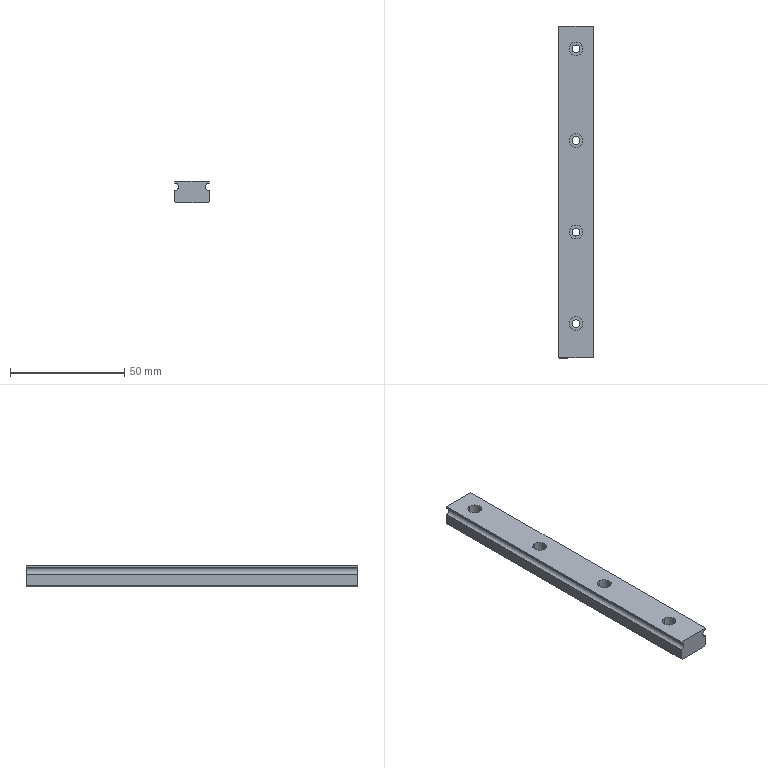Component | SolidWorks | 1-16-1 | 1 solid | 33 faces | box 15 x 145 x 9.5 mm | volume 18700 mm3 | cylinder 19 | plane 14 | commonest cylinder face diameters 6 x8 3.5 x8 3.28 x3
STEP:
#1=CARTESIAN_POINT('',(-4.34,3.239,-0.7858));
#2=VERTEX_POINT('',#1);
#3=CARTESIAN_POINT('',(-4.34,3.475,-0.7858));
#4=VERTEX_POINT('',#3);
#5=CARTESIAN_POINT('',(-4.34,3.357,-0.7858));
#6=DIRECTION('',(0.,0.,-1.));
#7=DIRECTION('',(0.,1.,0.));
#8=AXIS2_PLACEMENT_3D('',#5,#6,#7);
#9=CIRCLE('',#8,0.1181);
#10=EDGE_CURVE('',#2,#4,#9,.T.);
#11=ORIENTED_EDGE('',*,*,#10,.F.);
#12=CARTESIAN_POINT('',(-4.34,3.239,-0.963));
#13=VERTEX_POINT('',#12);
#14=CARTESIAN_POINT('',(-4.34,3.239,-0.8744));
#15=DIRECTION('',(0.,0.,-1.));
#16=VECTOR('',#15,39.37);
#17=LINE('',#14,#16);
#18=EDGE_CURVE('',#2,#13,#17,.T.);
#19=ORIENTED_EDGE('',*,*,#18,.T.);
#20=CARTESIAN_POINT('',(-4.34,3.475,-0.963));
#21=VERTEX_POINT('',#20);
#22=CARTESIAN_POINT('',(-4.34,3.357,-0.963));
#23=DIRECTION('',(-0.,-0.,1.));
#24=DIRECTION('',(0.,1.,0.));
#25=AXIS2_PLACEMENT_3D('',#22,#23,#24);
#26=CIRCLE('',#25,0.1181);
#27=EDGE_CURVE('',#21,#13,#26,.T.);
#28=ORIENTED_EDGE('',*,*,#27,.F.);
#29=CARTESIAN_POINT('',(-4.34,3.475,-0.8744));
#30=DIRECTION('',(0.,0.,-1.));
#31=VECTOR('',#30,39.37);
#32=LINE('',#29,#31);
#33=EDGE_CURVE('',#4,#21,#32,.T.);
#34=ORIENTED_EDGE('',*,*,#33,.F.);
#35=EDGE_LOOP('',(#11,#19,#28,#34));
#36=FACE_OUTER_BOUND('',#35,.T.);
#37=CARTESIAN_POINT('',(-4.34,3.357,-0.8744));
#38=DIRECTION('',(0.,0.,-1.));
#39=DIRECTION('',(0.,1.,0.));
#40=AXIS2_PLACEMENT_3D('',#37,#38,#39);
#41=CYLINDRICAL_SURFACE('',#40,0.1181);
#42=ADVANCED_FACE('',(#36),#41,.F.);
#43=CARTESIAN_POINT('',(-4.34,1.664,-0.7858));
#44=VERTEX_POINT('',#43);
#45=CARTESIAN_POINT('',(-4.34,1.9,-0.7858));
#46=VERTEX_POINT('',#45);
#47=CARTESIAN_POINT('',(-4.34,1.782,-0.7858));
#48=DIRECTION('',(0.,0.,-1.));
#49=DIRECTION('',(0.,1.,0.));
#50=AXIS2_PLACEMENT_3D('',#47,#48,#49);
#51=CIRCLE('',#50,0.1181);
#52=EDGE_CURVE('',#44,#46,#51,.T.);
#53=ORIENTED_EDGE('',*,*,#52,.F.);
#54=CARTESIAN_POINT('',(-4.34,1.664,-0.963));
#55=VERTEX_POINT('',#54);
#56=CARTESIAN_POINT('',(-4.34,1.664,-0.8744));
#57=DIRECTION('',(0.,0.,-1.));
#58=VECTOR('',#57,39.37);
#59=LINE('',#56,#58);
#60=EDGE_CURVE('',#44,#55,#59,.T.);
#61=ORIENTED_EDGE('',*,*,#60,.T.);
#62=CARTESIAN_POINT('',(-4.34,1.9,-0.963));
#63=VERTEX_POINT('',#62);
#64=CARTESIAN_POINT('',(-4.34,1.782,-0.963));
#65=DIRECTION('',(-0.,-0.,1.));
#66=DIRECTION('',(0.,1.,0.));
#67=AXIS2_PLACEMENT_3D('',#64,#65,#66);
#68=CIRCLE('',#67,0.1181);
#69=EDGE_CURVE('',#63,#55,#68,.T.);
#70=ORIENTED_EDGE('',*,*,#69,.F.);
#71=CARTESIAN_POINT('',(-4.34,1.9,-0.8744));
#72=DIRECTION('',(0.,0.,-1.));
#73=VECTOR('',#72,39.37);
#74=LINE('',#71,#73);
#75=EDGE_CURVE('',#46,#63,#74,.T.);
#76=ORIENTED_EDGE('',*,*,#75,.F.);
#77=EDGE_LOOP('',(#53,#61,#70,#76));
#78=FACE_OUTER_BOUND('',#77,.T.);
#79=CARTESIAN_POINT('',(-4.34,1.782,-0.8744));
#80=DIRECTION('',(0.,0.,-1.));
#81=DIRECTION('',(0.,1.,0.));
#82=AXIS2_PLACEMENT_3D('',#79,#80,#81);
#83=CYLINDRICAL_SURFACE('',#82,0.1181);
#84=ADVANCED_FACE('',(#78),#83,.F.);
#85=CARTESIAN_POINT('',(-4.34,6.389,-0.7858));
#86=VERTEX_POINT('',#85);
#87=CARTESIAN_POINT('',(-4.34,6.625,-0.7858));
#88=VERTEX_POINT('',#87);
#89=CARTESIAN_POINT('',(-4.34,6.507,-0.7858));
#90=DIRECTION('',(0.,0.,-1.));
#91=DIRECTION('',(0.,1.,0.));
#92=AXIS2_PLACEMENT_3D('',#89,#90,#91);
#93=CIRCLE('',#92,0.1181);
#94=EDGE_CURVE('',#86,#88,#93,.T.);
#95=ORIENTED_EDGE('',*,*,#94,.F.);
#96=CARTESIAN_POINT('',(-4.34,6.389,-0.963));
#97=VERTEX_POINT('',#96);
#98=CARTESIAN_POINT('',(-4.34,6.389,-0.8744));
#99=DIRECTION('',(0.,0.,-1.));
#100=VECTOR('',#99,39.37);
#101=LINE('',#98,#100);
#102=EDGE_CURVE('',#86,#97,#101,.T.);
#103=ORIENTED_EDGE('',*,*,#102,.T.);
#104=CARTESIAN_POINT('',(-4.34,6.625,-0.963));
#105=VERTEX_POINT('',#104);
#106=CARTESIAN_POINT('',(-4.34,6.507,-0.963));
#107=DIRECTION('',(-0.,-0.,1.));
#108=DIRECTION('',(0.,1.,0.));
#109=AXIS2_PLACEMENT_3D('',#106,#107,#108);
#110=CIRCLE('',#109,0.1181);
#111=EDGE_CURVE('',#105,#97,#110,.T.);
#112=ORIENTED_EDGE('',*,*,#111,.F.);
#113=CARTESIAN_POINT('',(-4.34,6.625,-0.8744));
#114=DIRECTION('',(0.,0.,-1.));
#115=VECTOR('',#114,39.37);
#116=LINE('',#113,#115);
#117=EDGE_CURVE('',#88,#105,#116,.T.);
#118=ORIENTED_EDGE('',*,*,#117,.F.);
#119=EDGE_LOOP('',(#95,#103,#112,#118));
#120=FACE_OUTER_BOUND('',#119,.T.);
#121=CARTESIAN_POINT('',(-4.34,6.507,-0.8744));
#122=DIRECTION('',(0.,0.,-1.));
#123=DIRECTION('',(0.,1.,0.));
#124=AXIS2_PLACEMENT_3D('',#121,#122,#123);
#125=CYLINDRICAL_SURFACE('',#124,0.1181);
#126=ADVANCED_FACE('',(#120),#125,.F.);
#127=CARTESIAN_POINT('',(-4.34,4.814,-0.7858));
#128=VERTEX_POINT('',#127);
#129=CARTESIAN_POINT('',(-4.34,5.05,-0.7858));
#130=VERTEX_POINT('',#129);
#131=CARTESIAN_POINT('',(-4.34,4.932,-0.7858));
#132=DIRECTION('',(0.,0.,-1.));
#133=DIRECTION('',(0.,1.,0.));
#134=AXIS2_PLACEMENT_3D('',#131,#132,#133);
#135=CIRCLE('',#134,0.1181);
#136=EDGE_CURVE('',#128,#130,#135,.T.);
#137=ORIENTED_EDGE('',*,*,#136,.F.);
#138=CARTESIAN_POINT('',(-4.34,4.814,-0.963));
#139=VERTEX_POINT('',#138);
#140=CARTESIAN_POINT('',(-4.34,4.814,-0.8744));
#141=DIRECTION('',(0.,0.,-1.));
#142=VECTOR('',#141,39.37);
#143=LINE('',#140,#142);
#144=EDGE_CURVE('',#128,#139,#143,.T.);
#145=ORIENTED_EDGE('',*,*,#144,.T.);
#146=CARTESIAN_POINT('',(-4.34,5.05,-0.963));
#147=VERTEX_POINT('',#146);
#148=CARTESIAN_POINT('',(-4.34,4.932,-0.963));
#149=DIRECTION('',(-0.,-0.,1.));
#150=DIRECTION('',(0.,1.,0.));
#151=AXIS2_PLACEMENT_3D('',#148,#149,#150);
#152=CIRCLE('',#151,0.1181);
#153=EDGE_CURVE('',#147,#139,#152,.T.);
#154=ORIENTED_EDGE('',*,*,#153,.F.);
#155=CARTESIAN_POINT('',(-4.34,5.05,-0.8744));
#156=DIRECTION('',(0.,0.,-1.));
#157=VECTOR('',#156,39.37);
#158=LINE('',#155,#157);
#159=EDGE_CURVE('',#130,#147,#158,.T.);
#160=ORIENTED_EDGE('',*,*,#159,.F.);
#161=EDGE_LOOP('',(#137,#145,#154,#160));
#162=FACE_OUTER_BOUND('',#161,.T.);
#163=CARTESIAN_POINT('',(-4.34,4.932,-0.8744));
#164=DIRECTION('',(0.,0.,-1.));
#165=DIRECTION('',(0.,1.,0.));
#166=AXIS2_PLACEMENT_3D('',#163,#164,#165);
#167=CYLINDRICAL_SURFACE('',#166,0.1181);
#168=ADVANCED_FACE('',(#162),#167,.F.);
#169=CARTESIAN_POINT('',(-4.11,1.192,-0.8834));
#170=VERTEX_POINT('',#169);
#171=CARTESIAN_POINT('',(-4.045,1.192,-0.8189));
#172=VERTEX_POINT('',#171);
#173=CARTESIAN_POINT('',(-4.045,1.192,-0.8834));
#174=DIRECTION('',(0.,1.,0.));
#175=DIRECTION('',(-1.,0.,0.));
#176=AXIS2_PLACEMENT_3D('',#173,#174,#175);
#177=CIRCLE('',#176,0.06457);
#178=EDGE_CURVE('',#170,#172,#177,.T.);
#179=ORIENTED_EDGE('',*,*,#178,.F.);
#180=CARTESIAN_POINT('',(-4.11,6.9,-0.8834));
#181=VERTEX_POINT('',#180);
#182=CARTESIAN_POINT('',(-4.11,7.097,-0.8834));
#183=DIRECTION('',(0.,1.,0.));
#184=VECTOR('',#183,39.37);
#185=LINE('',#182,#184);
#186=EDGE_CURVE('',#170,#181,#185,.T.);
#187=ORIENTED_EDGE('',*,*,#186,.T.);
#188=CARTESIAN_POINT('',(-4.045,6.9,-0.8189));
#189=VERTEX_POINT('',#188);
#190=CARTESIAN_POINT('',(-4.045,6.9,-0.8834));
#191=DIRECTION('',(-0.,-1.,-0.));
#192=DIRECTION('',(-1.,0.,0.));
#193=AXIS2_PLACEMENT_3D('',#190,#191,#192);
#194=CIRCLE('',#193,0.06457);
#195=EDGE_CURVE('',#189,#181,#194,.T.);
#196=ORIENTED_EDGE('',*,*,#195,.F.);
#197=CARTESIAN_POINT('',(-4.045,7.097,-0.8189));
#198=DIRECTION('',(0.,1.,0.));
#199=VECTOR('',#198,39.37);
#200=LINE('',#197,#199);
#201=EDGE_CURVE('',#172,#189,#200,.T.);
#202=ORIENTED_EDGE('',*,*,#201,.F.);
#203=EDGE_LOOP('',(#179,#187,#196,#202));
#204=FACE_OUTER_BOUND('',#203,.T.);
#205=CARTESIAN_POINT('',(-4.045,7.097,-0.8834));
#206=DIRECTION('',(0.,1.,0.));
#207=DIRECTION('',(-1.,0.,0.));
#208=AXIS2_PLACEMENT_3D('',#205,#206,#207);
#209=CYLINDRICAL_SURFACE('',#208,0.06457);
#210=ADVANCED_FACE('',(#204),#209,.F.);
#211=CARTESIAN_POINT('',(-4.34,3.288,-0.963));
#212=VERTEX_POINT('',#211);
#213=CARTESIAN_POINT('',(-4.34,3.426,-0.963));
#214=VERTEX_POINT('',#213);
#215=CARTESIAN_POINT('',(-4.34,3.357,-0.963));
#216=DIRECTION('',(0.,0.,-1.));
#217=DIRECTION('',(0.,1.,0.));
#218=AXIS2_PLACEMENT_3D('',#215,#216,#217);
#219=CIRCLE('',#218,0.0689);
#220=EDGE_CURVE('',#212,#214,#219,.T.);
#221=ORIENTED_EDGE('',*,*,#220,.F.);
#222=CARTESIAN_POINT('',(-4.34,3.288,-1.16));
#223=VERTEX_POINT('',#222);
#224=CARTESIAN_POINT('',(-4.34,3.288,-1.061));
#225=DIRECTION('',(0.,0.,-1.));
#226=VECTOR('',#225,39.37);
#227=LINE('',#224,#226);
#228=EDGE_CURVE('',#212,#223,#227,.T.);
#229=ORIENTED_EDGE('',*,*,#228,.T.);
#230=CARTESIAN_POINT('',(-4.34,3.426,-1.16));
#231=VERTEX_POINT('',#230);
#232=CARTESIAN_POINT('',(-4.34,3.357,-1.16));
#233=DIRECTION('',(-0.,-0.,1.));
#234=DIRECTION('',(0.,1.,0.));
#235=AXIS2_PLACEMENT_3D('',#232,#233,#234);
#236=CIRCLE('',#235,0.0689);
#237=EDGE_CURVE('',#231,#223,#236,.T.);
#238=ORIENTED_EDGE('',*,*,#237,.F.);
#239=CARTESIAN_POINT('',(-4.34,3.426,-1.061));
#240=DIRECTION('',(0.,0.,-1.));
#241=VECTOR('',#240,39.37);
#242=LINE('',#239,#241);
#243=EDGE_CURVE('',#214,#231,#242,.T.);
#244=ORIENTED_EDGE('',*,*,#243,.F.);
#245=EDGE_LOOP('',(#221,#229,#238,#244));
#246=FACE_OUTER_BOUND('',#245,.T.);
#247=CARTESIAN_POINT('',(-4.34,3.357,-1.061));
#248=DIRECTION('',(0.,0.,-1.));
#249=DIRECTION('',(0.,1.,0.));
#250=AXIS2_PLACEMENT_3D('',#247,#248,#249);
#251=CYLINDRICAL_SURFACE('',#250,0.0689);
#252=ADVANCED_FACE('',(#246),#251,.F.);
#253=CARTESIAN_POINT('',(-4.34,1.713,-0.963));
#254=VERTEX_POINT('',#253);
#255=CARTESIAN_POINT('',(-4.34,1.851,-0.963));
#256=VERTEX_POINT('',#255);
#257=CARTESIAN_POINT('',(-4.34,1.782,-0.963));
#258=DIRECTION('',(0.,0.,-1.));
#259=DIRECTION('',(0.,1.,0.));
#260=AXIS2_PLACEMENT_3D('',#257,#258,#259);
#261=CIRCLE('',#260,0.0689);
#262=EDGE_CURVE('',#254,#256,#261,.T.);
#263=ORIENTED_EDGE('',*,*,#262,.F.);
#264=CARTESIAN_POINT('',(-4.34,1.713,-1.16));
#265=VERTEX_POINT('',#264);
#266=CARTESIAN_POINT('',(-4.34,1.713,-1.061));
#267=DIRECTION('',(0.,0.,-1.));
#268=VECTOR('',#267,39.37);
#269=LINE('',#266,#268);
#270=EDGE_CURVE('',#254,#265,#269,.T.);
#271=ORIENTED_EDGE('',*,*,#270,.T.);
#272=CARTESIAN_POINT('',(-4.34,1.851,-1.16));
#273=VERTEX_POINT('',#272);
#274=CARTESIAN_POINT('',(-4.34,1.782,-1.16));
#275=DIRECTION('',(-0.,-0.,1.));
#276=DIRECTION('',(0.,1.,0.));
#277=AXIS2_PLACEMENT_3D('',#274,#275,#276);
#278=CIRCLE('',#277,0.0689);
#279=EDGE_CURVE('',#273,#265,#278,.T.);
#280=ORIENTED_EDGE('',*,*,#279,.F.);
#281=CARTESIAN_POINT('',(-4.34,1.851,-1.061));
#282=DIRECTION('',(0.,0.,-1.));
#283=VECTOR('',#282,39.37);
#284=LINE('',#281,#283);
#285=EDGE_CURVE('',#256,#273,#284,.T.);
#286=ORIENTED_EDGE('',*,*,#285,.F.);
#287=EDGE_LOOP('',(#263,#271,#280,#286));
#288=FACE_OUTER_BOUND('',#287,.T.);
#289=CARTESIAN_POINT('',(-4.34,1.782,-1.061));
#290=DIRECTION('',(0.,0.,-1.));
#291=DIRECTION('',(0.,1.,0.));
#292=AXIS2_PLACEMENT_3D('',#289,#290,#291);
#293=CYLINDRICAL_SURFACE('',#292,0.0689);
#294=ADVANCED_FACE('',(#288),#293,.F.);
#295=CARTESIAN_POINT('',(-4.34,6.438,-0.963));
#296=VERTEX_POINT('',#295);
#297=CARTESIAN_POINT('',(-4.34,6.576,-0.963));
#298=VERTEX_POINT('',#297);
#299=CARTESIAN_POINT('',(-4.34,6.507,-0.963));
#300=DIRECTION('',(0.,0.,-1.));
#301=DIRECTION('',(0.,1.,0.));
#302=AXIS2_PLACEMENT_3D('',#299,#300,#301);
#303=CIRCLE('',#302,0.0689);
#304=EDGE_CURVE('',#296,#298,#303,.T.);
#305=ORIENTED_EDGE('',*,*,#304,.F.);
#306=CARTESIAN_POINT('',(-4.34,6.438,-1.16));
#307=VERTEX_POINT('',#306);
#308=CARTESIAN_POINT('',(-4.34,6.438,-1.061));
#309=DIRECTION('',(0.,0.,-1.));
#310=VECTOR('',#309,39.37);
#311=LINE('',#308,#310);
#312=EDGE_CURVE('',#296,#307,#311,.T.);
#313=ORIENTED_EDGE('',*,*,#312,.T.);
#314=CARTESIAN_POINT('',(-4.34,6.576,-1.16));
#315=VERTEX_POINT('',#314);
#316=CARTESIAN_POINT('',(-4.34,6.507,-1.16));
#317=DIRECTION('',(-0.,-0.,1.));
#318=DIRECTION('',(0.,1.,0.));
#319=AXIS2_PLACEMENT_3D('',#316,#317,#318);
#320=CIRCLE('',#319,0.0689);
#321=EDGE_CURVE('',#315,#307,#320,.T.);
#322=ORIENTED_EDGE('',*,*,#321,.F.);
#323=CARTESIAN_POINT('',(-4.34,6.576,-1.061));
#324=DIRECTION('',(0.,0.,-1.));
#325=VECTOR('',#324,39.37);
#326=LINE('',#323,#325);
#327=EDGE_CURVE('',#298,#315,#326,.T.);
#328=ORIENTED_EDGE('',*,*,#327,.F.);
#329=EDGE_LOOP('',(#305,#313,#322,#328));
#330=FACE_OUTER_BOUND('',#329,.T.);
#331=CARTESIAN_POINT('',(-4.34,6.507,-1.061));
#332=DIRECTION('',(0.,0.,-1.));
#333=DIRECTION('',(0.,1.,0.));
#334=AXIS2_PLACEMENT_3D('',#331,#332,#333);
#335=CYLINDRICAL_SURFACE('',#334,0.0689);
#336=ADVANCED_FACE('',(#330),#335,.F.);
#337=CARTESIAN_POINT('',(-4.34,4.863,-0.963));
#338=VERTEX_POINT('',#337);
#339=CARTESIAN_POINT('',(-4.34,5.001,-0.963));
#340=VERTEX_POINT('',#339);
#341=CARTESIAN_POINT('',(-4.34,4.932,-0.963));
#342=DIRECTION('',(0.,0.,-1.));
#343=DIRECTION('',(0.,1.,0.));
#344=AXIS2_PLACEMENT_3D('',#341,#342,#343);
#345=CIRCLE('',#344,0.0689);
#346=EDGE_CURVE('',#338,#340,#345,.T.);
#347=ORIENTED_EDGE('',*,*,#346,.F.);
#348=CARTESIAN_POINT('',(-4.34,4.863,-1.16));
#349=VERTEX_POINT('',#348);
#350=CARTESIAN_POINT('',(-4.34,4.863,-1.061));
#351=DIRECTION('',(0.,0.,-1.));
#352=VECTOR('',#351,39.37);
#353=LINE('',#350,#352);
#354=EDGE_CURVE('',#338,#349,#353,.T.);
#355=ORIENTED_EDGE('',*,*,#354,.T.);
#356=CARTESIAN_POINT('',(-4.34,5.001,-1.16));
#357=VERTEX_POINT('',#356);
#358=CARTESIAN_POINT('',(-4.34,4.932,-1.16));
#359=DIRECTION('',(-0.,-0.,1.));
#360=DIRECTION('',(0.,1.,0.));
#361=AXIS2_PLACEMENT_3D('',#358,#359,#360);
#362=CIRCLE('',#361,0.0689);
#363=EDGE_CURVE('',#357,#349,#362,.T.);
#364=ORIENTED_EDGE('',*,*,#363,.F.);
#365=CARTESIAN_POINT('',(-4.34,5.001,-1.061));
#366=DIRECTION('',(0.,0.,-1.));
#367=VECTOR('',#366,39.37);
#368=LINE('',#365,#367);
#369=EDGE_CURVE('',#340,#357,#368,.T.);
#370=ORIENTED_EDGE('',*,*,#369,.F.);
#371=EDGE_LOOP('',(#347,#355,#364,#370));
#372=FACE_OUTER_BOUND('',#371,.T.);
#373=CARTESIAN_POINT('',(-4.34,4.932,-1.061));
#374=DIRECTION('',(0.,0.,-1.));
#375=DIRECTION('',(0.,1.,0.));
#376=AXIS2_PLACEMENT_3D('',#373,#374,#375);
#377=CYLINDRICAL_SURFACE('',#376,0.0689);
#378=ADVANCED_FACE('',(#372),#377,.F.);
#379=CARTESIAN_POINT('',(-4.636,1.192,-0.7858));
#380=VERTEX_POINT('',#379);
#381=CARTESIAN_POINT('',(-4.045,1.192,-0.7858));
#382=VERTEX_POINT('',#381);
#383=CARTESIAN_POINT('',(-4.636,1.192,-0.7858));
#384=DIRECTION('',(1.,-0.,0.));
#385=VECTOR('',#384,39.37);
#386=LINE('',#383,#385);
#387=EDGE_CURVE('',#380,#382,#386,.T.);
#388=ORIENTED_EDGE('',*,*,#387,.T.);
#389=CARTESIAN_POINT('',(-4.045,6.9,-0.7858));
#390=VERTEX_POINT('',#389);
#391=CARTESIAN_POINT('',(-4.045,7.097,-0.7858));
#392=DIRECTION('',(0.,1.,0.));
#393=VECTOR('',#392,39.37);
#394=LINE('',#391,#393);
#395=EDGE_CURVE('',#382,#390,#394,.T.);
#396=ORIENTED_EDGE('',*,*,#395,.T.);
#397=CARTESIAN_POINT('',(-4.636,6.9,-0.7858));
#398=VERTEX_POINT('',#397);
#399=CARTESIAN_POINT('',(-4.636,6.9,-0.7858));
#400=DIRECTION('',(-1.,0.,-0.));
#401=VECTOR('',#400,39.37);
#402=LINE('',#399,#401);
#403=EDGE_CURVE('',#390,#398,#402,.T.);
#404=ORIENTED_EDGE('',*,*,#403,.T.);
#405=CARTESIAN_POINT('',(-4.636,7.097,-0.7858));
#406=DIRECTION('',(-0.,-1.,-0.));
#407=VECTOR('',#406,39.37);
#408=LINE('',#405,#407);
#409=EDGE_CURVE('',#398,#380,#408,.T.);
#410=ORIENTED_EDGE('',*,*,#409,.T.);
#411=EDGE_LOOP('',(#388,#396,#404,#410));
#412=FACE_OUTER_BOUND('',#411,.T.);
#413=CARTESIAN_POINT('',(-4.34,3.357,-0.7858));
#414=DIRECTION('',(0.,0.,-1.));
#415=DIRECTION('',(0.,1.,0.));
#416=AXIS2_PLACEMENT_3D('',#413,#414,#415);
#417=CIRCLE('',#416,0.1181);
#418=EDGE_CURVE('',#4,#2,#417,.T.);
#419=ORIENTED_EDGE('',*,*,#418,.T.);
#420=ORIENTED_EDGE('',*,*,#10,.T.);
#421=EDGE_LOOP('',(#419,#420));
#422=FACE_BOUND('',#421,.T.);
#423=CARTESIAN_POINT('',(-4.34,1.782,-0.7858));
#424=DIRECTION('',(0.,0.,-1.));
#425=DIRECTION('',(0.,1.,0.));
#426=AXIS2_PLACEMENT_3D('',#423,#424,#425);
#427=CIRCLE('',#426,0.1181);
#428=EDGE_CURVE('',#46,#44,#427,.T.);
#429=ORIENTED_EDGE('',*,*,#428,.T.);
#430=ORIENTED_EDGE('',*,*,#52,.T.);
#431=EDGE_LOOP('',(#429,#430));
#432=FACE_BOUND('',#431,.T.);
#433=CARTESIAN_POINT('',(-4.34,6.507,-0.7858));
#434=DIRECTION('',(0.,0.,-1.));
#435=DIRECTION('',(0.,1.,0.));
#436=AXIS2_PLACEMENT_3D('',#433,#434,#435);
#437=CIRCLE('',#436,0.1181);
#438=EDGE_CURVE('',#88,#86,#437,.T.);
#439=ORIENTED_EDGE('',*,*,#438,.T.);
#440=ORIENTED_EDGE('',*,*,#94,.T.);
#441=EDGE_LOOP('',(#439,#440));
#442=FACE_BOUND('',#441,.T.);
#443=CARTESIAN_POINT('',(-4.34,4.932,-0.7858));
#444=DIRECTION('',(0.,0.,-1.));
#445=DIRECTION('',(0.,1.,0.));
#446=AXIS2_PLACEMENT_3D('',#443,#444,#445);
#447=CIRCLE('',#446,0.1181);
#448=EDGE_CURVE('',#130,#128,#447,.T.);
#449=ORIENTED_EDGE('',*,*,#448,.T.);
#450=ORIENTED_EDGE('',*,*,#136,.T.);
#451=EDGE_LOOP('',(#449,#450));
#452=FACE_BOUND('',#451,.T.);
#453=CARTESIAN_POINT('',(-4.636,7.097,-0.7858));
#454=DIRECTION('',(-0.,-0.,1.));
#455=DIRECTION('',(-0.,-1.,-0.));
#456=AXIS2_PLACEMENT_3D('',#453,#454,#455);
#457=PLANE('',#456);
#458=ADVANCED_FACE('',(#412,#422,#432,#442,#452),#457,.T.);
#459=CARTESIAN_POINT('',(-4.045,1.192,-0.7858));
#460=DIRECTION('',(0.,0.,-1.));
#461=VECTOR('',#460,39.37);
#462=LINE('',#459,#461);
#463=EDGE_CURVE('',#382,#172,#462,.T.);
#464=ORIENTED_EDGE('',*,*,#463,.T.);
#465=ORIENTED_EDGE('',*,*,#201,.T.);
#466=CARTESIAN_POINT('',(-4.045,6.9,-0.7858));
#467=DIRECTION('',(-0.,-0.,1.));
#468=VECTOR('',#467,39.37);
#469=LINE('',#466,#468);
#470=EDGE_CURVE('',#189,#390,#469,.T.);
#471=ORIENTED_EDGE('',*,*,#470,.T.);
#472=ORIENTED_EDGE('',*,*,#395,.F.);
#473=EDGE_LOOP('',(#464,#465,#471,#472));
#474=FACE_OUTER_BOUND('',#473,.T.);
#475=CARTESIAN_POINT('',(-4.045,7.097,-0.7858));
#476=DIRECTION('',(1.,-0.,0.));
#477=DIRECTION('',(0.,1.,0.));
#478=AXIS2_PLACEMENT_3D('',#475,#476,#477);
#479=PLANE('',#478);
#480=ADVANCED_FACE('',(#474),#479,.T.);
#481=CARTESIAN_POINT('',(-4.045,1.192,-1.14));
#482=VERTEX_POINT('',#481);
#483=CARTESIAN_POINT('',(-4.065,1.192,-1.16));
#484=VERTEX_POINT('',#483);
#485=CARTESIAN_POINT('',(-4.045,1.192,-1.14));
#486=DIRECTION('',(-0.7071,0.,-0.7071));
#487=VECTOR('',#486,39.37);
#488=LINE('',#485,#487);
#489=EDGE_CURVE('',#482,#484,#488,.T.);
#490=ORIENTED_EDGE('',*,*,#489,.F.);
#491=CARTESIAN_POINT('',(-4.045,1.192,-0.948));
#492=VERTEX_POINT('',#491);
#493=CARTESIAN_POINT('',(-4.045,1.192,-1.16));
#494=DIRECTION('',(-0.,-0.,1.));
#495=VECTOR('',#494,39.37);
#496=LINE('',#493,#495);
#497=EDGE_CURVE('',#482,#492,#496,.T.);
#498=ORIENTED_EDGE('',*,*,#497,.T.);
#499=CARTESIAN_POINT('',(-4.045,1.192,-0.8834));
#500=DIRECTION('',(0.,1.,0.));
#501=DIRECTION('',(-1.,0.,0.));
#502=AXIS2_PLACEMENT_3D('',#499,#500,#501);
#503=CIRCLE('',#502,0.06457);
#504=EDGE_CURVE('',#492,#170,#503,.T.);
#505=ORIENTED_EDGE('',*,*,#504,.T.);
#506=ORIENTED_EDGE('',*,*,#178,.T.);
#507=ORIENTED_EDGE('',*,*,#463,.F.);
#508=ORIENTED_EDGE('',*,*,#387,.F.);
#509=CARTESIAN_POINT('',(-4.636,1.192,-0.8189));
#510=VERTEX_POINT('',#509);
#511=CARTESIAN_POINT('',(-4.636,1.192,-1.16));
#512=DIRECTION('',(0.,0.,-1.));
#513=VECTOR('',#512,39.37);
#514=LINE('',#511,#513);
#515=EDGE_CURVE('',#380,#510,#514,.T.);
#516=ORIENTED_EDGE('',*,*,#515,.T.);
#517=CARTESIAN_POINT('',(-4.636,1.192,-0.948));
#518=VERTEX_POINT('',#517);
#519=CARTESIAN_POINT('',(-4.636,1.192,-0.8834));
#520=DIRECTION('',(0.,1.,0.));
#521=DIRECTION('',(-1.,0.,0.));
#522=AXIS2_PLACEMENT_3D('',#519,#520,#521);
#523=CIRCLE('',#522,0.06457);
#524=EDGE_CURVE('',#510,#518,#523,.T.);
#525=ORIENTED_EDGE('',*,*,#524,.T.);
#526=CARTESIAN_POINT('',(-4.636,1.192,-1.14));
#527=VERTEX_POINT('',#526);
#528=CARTESIAN_POINT('',(-4.636,1.192,-1.16));
#529=DIRECTION('',(0.,0.,-1.));
#530=VECTOR('',#529,39.37);
#531=LINE('',#528,#530);
#532=EDGE_CURVE('',#518,#527,#531,.T.);
#533=ORIENTED_EDGE('',*,*,#532,.T.);
#534=CARTESIAN_POINT('',(-4.616,1.192,-1.16));
#535=VERTEX_POINT('',#534);
#536=CARTESIAN_POINT('',(-4.616,1.192,-1.16));
#537=DIRECTION('',(-0.7071,0.,0.7071));
#538=VECTOR('',#537,39.37);
#539=LINE('',#536,#538);
#540=EDGE_CURVE('',#535,#527,#539,.T.);
#541=ORIENTED_EDGE('',*,*,#540,.F.);
#542=CARTESIAN_POINT('',(-4.34,1.192,-1.16));
#543=DIRECTION('',(1.,-0.,0.));
#544=VECTOR('',#543,39.37);
#545=LINE('',#542,#544);
#546=EDGE_CURVE('',#535,#484,#545,.T.);
#547=ORIENTED_EDGE('',*,*,#546,.T.);
#548=EDGE_LOOP('',(#490,#498,#505,#506,#507,#508,#516,#525,#533,#541,#547));
#549=FACE_OUTER_BOUND('',#548,.T.);
#550=CARTESIAN_POINT('',(-4.34,1.192,-1.16));
#551=DIRECTION('',(-0.,-1.,-0.));
#552=DIRECTION('',(1.,-0.,0.));
#553=AXIS2_PLACEMENT_3D('',#550,#551,#552);
#554=PLANE('',#553);
#555=ADVANCED_FACE('',(#549),#554,.T.);
#556=ORIENTED_EDGE('',*,*,#515,.F.);
#557=ORIENTED_EDGE('',*,*,#409,.F.);
#558=CARTESIAN_POINT('',(-4.636,6.9,-0.8189));
#559=VERTEX_POINT('',#558);
#560=CARTESIAN_POINT('',(-4.636,6.9,-0.8189));
#561=DIRECTION('',(0.,0.,-1.));
#562=VECTOR('',#561,39.37);
#563=LINE('',#560,#562);
#564=EDGE_CURVE('',#398,#559,#563,.T.);
#565=ORIENTED_EDGE('',*,*,#564,.T.);
#566=CARTESIAN_POINT('',(-4.636,7.097,-0.8189));
#567=DIRECTION('',(-0.,-1.,-0.));
#568=VECTOR('',#567,39.37);
#569=LINE('',#566,#568);
#570=EDGE_CURVE('',#559,#510,#569,.T.);
#571=ORIENTED_EDGE('',*,*,#570,.T.);
#572=EDGE_LOOP('',(#556,#557,#565,#571));
#573=FACE_OUTER_BOUND('',#572,.T.);
#574=CARTESIAN_POINT('',(-4.636,7.097,-0.8189));
#575=DIRECTION('',(-1.,0.,-0.));
#576=DIRECTION('',(-0.,-1.,-0.));
#577=AXIS2_PLACEMENT_3D('',#574,#575,#576);
#578=PLANE('',#577);
#579=ADVANCED_FACE('',(#573),#578,.T.);
#580=CARTESIAN_POINT('',(-4.065,6.9,-1.16));
#581=VERTEX_POINT('',#580);
#582=CARTESIAN_POINT('',(-4.616,6.9,-1.16));
#583=VERTEX_POINT('',#582);
#584=CARTESIAN_POINT('',(-4.34,6.9,-1.16));
#585=DIRECTION('',(-1.,0.,-0.));
#586=VECTOR('',#585,39.37);
#587=LINE('',#584,#586);
#588=EDGE_CURVE('',#581,#583,#587,.T.);
#589=ORIENTED_EDGE('',*,*,#588,.T.);
#590=CARTESIAN_POINT('',(-4.636,6.9,-1.14));
#591=VERTEX_POINT('',#590);
#592=CARTESIAN_POINT('',(-4.616,6.9,-1.16));
#593=DIRECTION('',(0.7071,-0.,-0.7071));
#594=VECTOR('',#593,39.37);
#595=LINE('',#592,#594);
#596=EDGE_CURVE('',#591,#583,#595,.T.);
#597=ORIENTED_EDGE('',*,*,#596,.F.);
#598=CARTESIAN_POINT('',(-4.636,6.9,-0.948));
#599=VERTEX_POINT('',#598);
#600=CARTESIAN_POINT('',(-4.636,6.9,-1.16));
#601=DIRECTION('',(-0.,-0.,1.));
#602=VECTOR('',#601,39.37);
#603=LINE('',#600,#602);
#604=EDGE_CURVE('',#591,#599,#603,.T.);
#605=ORIENTED_EDGE('',*,*,#604,.T.);
#606=CARTESIAN_POINT('',(-4.636,6.9,-0.8834));
#607=DIRECTION('',(-0.,-1.,-0.));
#608=DIRECTION('',(-1.,0.,0.));
#609=AXIS2_PLACEMENT_3D('',#606,#607,#608);
#610=CIRCLE('',#609,0.06457);
#611=EDGE_CURVE('',#599,#559,#610,.T.);
#612=ORIENTED_EDGE('',*,*,#611,.T.);
#613=ORIENTED_EDGE('',*,*,#564,.F.);
#614=ORIENTED_EDGE('',*,*,#403,.F.);
#615=ORIENTED_EDGE('',*,*,#470,.F.);
#616=ORIENTED_EDGE('',*,*,#195,.T.);
#617=CARTESIAN_POINT('',(-4.045,6.9,-0.948));
#618=VERTEX_POINT('',#617);
#619=CARTESIAN_POINT('',(-4.045,6.9,-0.8834));
#620=DIRECTION('',(-0.,-1.,-0.));
#621=DIRECTION('',(-1.,0.,0.));
#622=AXIS2_PLACEMENT_3D('',#619,#620,#621);
#623=CIRCLE('',#622,0.06457);
#624=EDGE_CURVE('',#181,#618,#623,.T.);
#625=ORIENTED_EDGE('',*,*,#624,.T.);
#626=CARTESIAN_POINT('',(-4.045,6.9,-1.14));
#627=VERTEX_POINT('',#626);
#628=CARTESIAN_POINT('',(-4.045,6.9,-1.16));
#629=DIRECTION('',(0.,0.,-1.));
#630=VECTOR('',#629,39.37);
#631=LINE('',#628,#630);
#632=EDGE_CURVE('',#618,#627,#631,.T.);
#633=ORIENTED_EDGE('',*,*,#632,.T.);
#634=CARTESIAN_POINT('',(-4.045,6.9,-1.14));
#635=DIRECTION('',(0.7071,-0.,0.7071));
#636=VECTOR('',#635,39.37);
#637=LINE('',#634,#636);
#638=EDGE_CURVE('',#581,#627,#637,.T.);
#639=ORIENTED_EDGE('',*,*,#638,.F.);
#640=EDGE_LOOP('',(#589,#597,#605,#612,#613,#614,#615,#616,#625,#633,#639));
#641=FACE_OUTER_BOUND('',#640,.T.);
#642=CARTESIAN_POINT('',(-4.34,6.9,-1.16));
#643=DIRECTION('',(0.,1.,0.));
#644=DIRECTION('',(-1.,0.,-0.));
#645=AXIS2_PLACEMENT_3D('',#642,#643,#644);
#646=PLANE('',#645);
#647=ADVANCED_FACE('',(#641),#646,.T.);
#648=ORIENTED_EDGE('',*,*,#18,.F.);
#649=ORIENTED_EDGE('',*,*,#418,.F.);
#650=ORIENTED_EDGE('',*,*,#33,.T.);
#651=CARTESIAN_POINT('',(-4.34,3.357,-0.963));
#652=DIRECTION('',(-0.,-0.,1.));
#653=DIRECTION('',(0.,1.,0.));
#654=AXIS2_PLACEMENT_3D('',#651,#652,#653);
#655=CIRCLE('',#654,0.1181);
#656=EDGE_CURVE('',#13,#21,#655,.T.);
#657=ORIENTED_EDGE('',*,*,#656,.F.);
#658=EDGE_LOOP('',(#648,#649,#650,#657));
#659=FACE_OUTER_BOUND('',#658,.T.);
#660=CARTESIAN_POINT('',(-4.34,3.357,-0.8744));
#661=DIRECTION('',(0.,0.,-1.));
#662=DIRECTION('',(0.,1.,0.));
#663=AXIS2_PLACEMENT_3D('',#660,#661,#662);
#664=CYLINDRICAL_SURFACE('',#663,0.1181);
#665=ADVANCED_FACE('',(#659),#664,.F.);
#666=ORIENTED_EDGE('',*,*,#60,.F.);
#667=ORIENTED_EDGE('',*,*,#428,.F.);
#668=ORIENTED_EDGE('',*,*,#75,.T.);
#669=CARTESIAN_POINT('',(-4.34,1.782,-0.963));
#670=DIRECTION('',(-0.,-0.,1.));
#671=DIRECTION('',(0.,1.,0.));
#672=AXIS2_PLACEMENT_3D('',#669,#670,#671);
#673=CIRCLE('',#672,0.1181);
#674=EDGE_CURVE('',#55,#63,#673,.T.);
#675=ORIENTED_EDGE('',*,*,#674,.F.);
#676=EDGE_LOOP('',(#666,#667,#668,#675));
#677=FACE_OUTER_BOUND('',#676,.T.);
#678=CARTESIAN_POINT('',(-4.34,1.782,-0.8744));
#679=DIRECTION('',(0.,0.,-1.));
#680=DIRECTION('',(0.,1.,0.));
#681=AXIS2_PLACEMENT_3D('',#678,#679,#680);
#682=CYLINDRICAL_SURFACE('',#681,0.1181);
#683=ADVANCED_FACE('',(#677),#682,.F.);
#684=ORIENTED_EDGE('',*,*,#102,.F.);
#685=ORIENTED_EDGE('',*,*,#438,.F.);
#686=ORIENTED_EDGE('',*,*,#117,.T.);
#687=CARTESIAN_POINT('',(-4.34,6.507,-0.963));
#688=DIRECTION('',(-0.,-0.,1.));
#689=DIRECTION('',(0.,1.,0.));
#690=AXIS2_PLACEMENT_3D('',#687,#688,#689);
#691=CIRCLE('',#690,0.1181);
#692=EDGE_CURVE('',#97,#105,#691,.T.);
#693=ORIENTED_EDGE('',*,*,#692,.F.);
#694=EDGE_LOOP('',(#684,#685,#686,#693));
#695=FACE_OUTER_BOUND('',#694,.T.);
#696=CARTESIAN_POINT('',(-4.34,6.507,-0.8744));
#697=DIRECTION('',(0.,0.,-1.));
#698=DIRECTION('',(0.,1.,0.));
#699=AXIS2_PLACEMENT_3D('',#696,#697,#698);
#700=CYLINDRICAL_SURFACE('',#699,0.1181);
#701=ADVANCED_FACE('',(#695),#700,.F.);
#702=ORIENTED_EDGE('',*,*,#144,.F.);
#703=ORIENTED_EDGE('',*,*,#448,.F.);
#704=ORIENTED_EDGE('',*,*,#159,.T.);
#705=CARTESIAN_POINT('',(-4.34,4.932,-0.963));
#706=DIRECTION('',(-0.,-0.,1.));
#707=DIRECTION('',(0.,1.,0.));
#708=AXIS2_PLACEMENT_3D('',#705,#706,#707);
#709=CIRCLE('',#708,0.1181);
#710=EDGE_CURVE('',#139,#147,#709,.T.);
#711=ORIENTED_EDGE('',*,*,#710,.F.);
#712=EDGE_LOOP('',(#702,#703,#704,#711));
#713=FACE_OUTER_BOUND('',#712,.T.);
#714=CARTESIAN_POINT('',(-4.34,4.932,-0.8744));
#715=DIRECTION('',(0.,0.,-1.));
#716=DIRECTION('',(0.,1.,0.));
#717=AXIS2_PLACEMENT_3D('',#714,#715,#716);
#718=CYLINDRICAL_SURFACE('',#717,0.1181);
#719=ADVANCED_FACE('',(#713),#718,.F.);
#720=ORIENTED_EDGE('',*,*,#186,.F.);
#721=ORIENTED_EDGE('',*,*,#504,.F.);
#722=CARTESIAN_POINT('',(-4.045,7.097,-0.948));
#723=DIRECTION('',(-0.,-1.,-0.));
#724=VECTOR('',#723,39.37);
#725=LINE('',#722,#724);
#726=EDGE_CURVE('',#618,#492,#725,.T.);
#727=ORIENTED_EDGE('',*,*,#726,.F.);
#728=ORIENTED_EDGE('',*,*,#624,.F.);
#729=EDGE_LOOP('',(#720,#721,#727,#728));
#730=FACE_OUTER_BOUND('',#729,.T.);
#731=CARTESIAN_POINT('',(-4.045,7.097,-0.8834));
#732=DIRECTION('',(0.,1.,0.));
#733=DIRECTION('',(-1.,0.,0.));
#734=AXIS2_PLACEMENT_3D('',#731,#732,#733);
#735=CYLINDRICAL_SURFACE('',#734,0.06457);
#736=ADVANCED_FACE('',(#730),#735,.F.);
#737=ORIENTED_EDGE('',*,*,#497,.F.);
#738=CARTESIAN_POINT('',(-4.045,7.097,-1.14));
#739=DIRECTION('',(0.,1.,0.));
#740=VECTOR('',#739,39.37);
#741=LINE('',#738,#740);
#742=EDGE_CURVE('',#482,#627,#741,.T.);
#743=ORIENTED_EDGE('',*,*,#742,.T.);
#744=ORIENTED_EDGE('',*,*,#632,.F.);
#745=ORIENTED_EDGE('',*,*,#726,.T.);
#746=EDGE_LOOP('',(#737,#743,#744,#745));
#747=FACE_OUTER_BOUND('',#746,.T.);
#748=CARTESIAN_POINT('',(-4.045,7.097,-0.948));
#749=DIRECTION('',(1.,-0.,0.));
#750=DIRECTION('',(0.,1.,0.));
#751=AXIS2_PLACEMENT_3D('',#748,#749,#750);
#752=PLANE('',#751);
#753=ADVANCED_FACE('',(#747),#752,.T.);
#754=ORIENTED_EDGE('',*,*,#546,.F.);
#755=CARTESIAN_POINT('',(-4.616,7.097,-1.16));
#756=DIRECTION('',(0.,1.,0.));
#757=VECTOR('',#756,39.37);
#758=LINE('',#755,#757);
#759=EDGE_CURVE('',#535,#583,#758,.T.);
#760=ORIENTED_EDGE('',*,*,#759,.T.);
#761=ORIENTED_EDGE('',*,*,#588,.F.);
#762=CARTESIAN_POINT('',(-4.065,7.097,-1.16));
#763=DIRECTION('',(-0.,-1.,-0.));
#764=VECTOR('',#763,39.37);
#765=LINE('',#762,#764);
#766=EDGE_CURVE('',#581,#484,#765,.T.);
#767=ORIENTED_EDGE('',*,*,#766,.T.);
#768=EDGE_LOOP('',(#754,#760,#761,#767));
#769=FACE_OUTER_BOUND('',#768,.T.);
#770=ORIENTED_EDGE('',*,*,#237,.T.);
#771=CARTESIAN_POINT('',(-4.34,3.357,-1.16));
#772=DIRECTION('',(-0.,-0.,1.));
#773=DIRECTION('',(0.,1.,0.));
#774=AXIS2_PLACEMENT_3D('',#771,#772,#773);
#775=CIRCLE('',#774,0.0689);
#776=EDGE_CURVE('',#223,#231,#775,.T.);
#777=ORIENTED_EDGE('',*,*,#776,.T.);
#778=EDGE_LOOP('',(#770,#777));
#779=FACE_BOUND('',#778,.T.);
#780=ORIENTED_EDGE('',*,*,#279,.T.);
#781=CARTESIAN_POINT('',(-4.34,1.782,-1.16));
#782=DIRECTION('',(-0.,-0.,1.));
#783=DIRECTION('',(0.,1.,0.));
#784=AXIS2_PLACEMENT_3D('',#781,#782,#783);
#785=CIRCLE('',#784,0.0689);
#786=EDGE_CURVE('',#265,#273,#785,.T.);
#787=ORIENTED_EDGE('',*,*,#786,.T.);
#788=EDGE_LOOP('',(#780,#787));
#789=FACE_BOUND('',#788,.T.);
#790=ORIENTED_EDGE('',*,*,#321,.T.);
#791=CARTESIAN_POINT('',(-4.34,6.507,-1.16));
#792=DIRECTION('',(-0.,-0.,1.));
#793=DIRECTION('',(0.,1.,0.));
#794=AXIS2_PLACEMENT_3D('',#791,#792,#793);
#795=CIRCLE('',#794,0.0689);
#796=EDGE_CURVE('',#307,#315,#795,.T.);
#797=ORIENTED_EDGE('',*,*,#796,.T.);
#798=EDGE_LOOP('',(#790,#797));
#799=FACE_BOUND('',#798,.T.);
#800=ORIENTED_EDGE('',*,*,#363,.T.);
#801=CARTESIAN_POINT('',(-4.34,4.932,-1.16));
#802=DIRECTION('',(-0.,-0.,1.));
#803=DIRECTION('',(0.,1.,0.));
#804=AXIS2_PLACEMENT_3D('',#801,#802,#803);
#805=CIRCLE('',#804,0.0689);
#806=EDGE_CURVE('',#349,#357,#805,.T.);
#807=ORIENTED_EDGE('',*,*,#806,.T.);
#808=EDGE_LOOP('',(#800,#807));
#809=FACE_BOUND('',#808,.T.);
#810=CARTESIAN_POINT('',(-4.065,7.097,-1.16));
#811=DIRECTION('',(0.,0.,-1.));
#812=DIRECTION('',(0.,1.,0.));
#813=AXIS2_PLACEMENT_3D('',#810,#811,#812);
#814=PLANE('',#813);
#815=ADVANCED_FACE('',(#769,#779,#789,#799,#809),#814,.T.);
#816=ORIENTED_EDGE('',*,*,#532,.F.);
#817=CARTESIAN_POINT('',(-4.636,7.097,-0.948));
#818=DIRECTION('',(0.,1.,0.));
#819=VECTOR('',#818,39.37);
#820=LINE('',#817,#819);
#821=EDGE_CURVE('',#518,#599,#820,.T.);
#822=ORIENTED_EDGE('',*,*,#821,.T.);
#823=ORIENTED_EDGE('',*,*,#604,.F.);
#824=CARTESIAN_POINT('',(-4.636,7.097,-1.14));
#825=DIRECTION('',(-0.,-1.,-0.));
#826=VECTOR('',#825,39.37);
#827=LINE('',#824,#826);
#828=EDGE_CURVE('',#591,#527,#827,.T.);
#829=ORIENTED_EDGE('',*,*,#828,.T.);
#830=EDGE_LOOP('',(#816,#822,#823,#829));
#831=FACE_OUTER_BOUND('',#830,.T.);
#832=CARTESIAN_POINT('',(-4.636,7.097,-1.14));
#833=DIRECTION('',(-1.,0.,-0.));
#834=DIRECTION('',(-0.,-1.,-0.));
#835=AXIS2_PLACEMENT_3D('',#832,#833,#834);
#836=PLANE('',#835);
#837=ADVANCED_FACE('',(#831),#836,.T.);
#838=ORIENTED_EDGE('',*,*,#821,.F.);
#839=ORIENTED_EDGE('',*,*,#524,.F.);
#840=ORIENTED_EDGE('',*,*,#570,.F.);
#841=ORIENTED_EDGE('',*,*,#611,.F.);
#842=EDGE_LOOP('',(#838,#839,#840,#841));
#843=FACE_OUTER_BOUND('',#842,.T.);
#844=CARTESIAN_POINT('',(-4.636,7.097,-0.8834));
#845=DIRECTION('',(0.,1.,0.));
#846=DIRECTION('',(-1.,0.,0.));
#847=AXIS2_PLACEMENT_3D('',#844,#845,#846);
#848=CYLINDRICAL_SURFACE('',#847,0.06457);
#849=ADVANCED_FACE('',(#843),#848,.F.);
#850=ORIENTED_EDGE('',*,*,#27,.T.);
#851=ORIENTED_EDGE('',*,*,#656,.T.);
#852=EDGE_LOOP('',(#850,#851));
#853=FACE_OUTER_BOUND('',#852,.T.);
#854=CARTESIAN_POINT('',(-4.34,3.357,-0.963));
#855=DIRECTION('',(0.,0.,-1.));
#856=DIRECTION('',(0.,1.,0.));
#857=AXIS2_PLACEMENT_3D('',#854,#855,#856);
#858=CIRCLE('',#857,0.0689);
#859=EDGE_CURVE('',#214,#212,#858,.T.);
#860=ORIENTED_EDGE('',*,*,#859,.T.);
#861=ORIENTED_EDGE('',*,*,#220,.T.);
#862=EDGE_LOOP('',(#860,#861));
#863=FACE_BOUND('',#862,.T.);
#864=CARTESIAN_POINT('',(-4.34,3.451,-0.963));
#865=DIRECTION('',(-0.,-0.,1.));
#866=DIRECTION('',(-0.,-1.,-0.));
#867=AXIS2_PLACEMENT_3D('',#864,#865,#866);
#868=PLANE('',#867);
#869=ADVANCED_FACE('',(#853,#863),#868,.T.);
#870=ORIENTED_EDGE('',*,*,#69,.T.);
#871=ORIENTED_EDGE('',*,*,#674,.T.);
#872=EDGE_LOOP('',(#870,#871));
#873=FACE_OUTER_BOUND('',#872,.T.);
#874=CARTESIAN_POINT('',(-4.34,1.782,-0.963));
#875=DIRECTION('',(0.,0.,-1.));
#876=DIRECTION('',(0.,1.,0.));
#877=AXIS2_PLACEMENT_3D('',#874,#875,#876);
#878=CIRCLE('',#877,0.0689);
#879=EDGE_CURVE('',#256,#254,#878,.T.);
#880=ORIENTED_EDGE('',*,*,#879,.T.);
#881=ORIENTED_EDGE('',*,*,#262,.T.);
#882=EDGE_LOOP('',(#880,#881));
#883=FACE_BOUND('',#882,.T.);
#884=CARTESIAN_POINT('',(-4.34,1.876,-0.963));
#885=DIRECTION('',(-0.,-0.,1.));
#886=DIRECTION('',(-0.,-1.,-0.));
#887=AXIS2_PLACEMENT_3D('',#884,#885,#886);
#888=PLANE('',#887);
#889=ADVANCED_FACE('',(#873,#883),#888,.T.);
#890=ORIENTED_EDGE('',*,*,#111,.T.);
#891=ORIENTED_EDGE('',*,*,#692,.T.);
#892=EDGE_LOOP('',(#890,#891));
#893=FACE_OUTER_BOUND('',#892,.T.);
#894=CARTESIAN_POINT('',(-4.34,6.507,-0.963));
#895=DIRECTION('',(0.,0.,-1.));
#896=DIRECTION('',(0.,1.,0.));
#897=AXIS2_PLACEMENT_3D('',#894,#895,#896);
#898=CIRCLE('',#897,0.0689);
#899=EDGE_CURVE('',#298,#296,#898,.T.);
#900=ORIENTED_EDGE('',*,*,#899,.T.);
#901=ORIENTED_EDGE('',*,*,#304,.T.);
#902=EDGE_LOOP('',(#900,#901));
#903=FACE_BOUND('',#902,.T.);
#904=CARTESIAN_POINT('',(-4.34,6.6,-0.963));
#905=DIRECTION('',(-0.,-0.,1.));
#906=DIRECTION('',(-0.,-1.,-0.));
#907=AXIS2_PLACEMENT_3D('',#904,#905,#906);
#908=PLANE('',#907);
#909=ADVANCED_FACE('',(#893,#903),#908,.T.);
#910=ORIENTED_EDGE('',*,*,#153,.T.);
#911=ORIENTED_EDGE('',*,*,#710,.T.);
#912=EDGE_LOOP('',(#910,#911));
#913=FACE_OUTER_BOUND('',#912,.T.);
#914=CARTESIAN_POINT('',(-4.34,4.932,-0.963));
#915=DIRECTION('',(0.,0.,-1.));
#916=DIRECTION('',(0.,1.,0.));
#917=AXIS2_PLACEMENT_3D('',#914,#915,#916);
#918=CIRCLE('',#917,0.0689);
#919=EDGE_CURVE('',#340,#338,#918,.T.);
#920=ORIENTED_EDGE('',*,*,#919,.T.);
#921=ORIENTED_EDGE('',*,*,#346,.T.);
#922=EDGE_LOOP('',(#920,#921));
#923=FACE_BOUND('',#922,.T.);
#924=CARTESIAN_POINT('',(-4.34,5.025,-0.963));
#925=DIRECTION('',(-0.,-0.,1.));
#926=DIRECTION('',(-0.,-1.,-0.));
#927=AXIS2_PLACEMENT_3D('',#924,#925,#926);
#928=PLANE('',#927);
#929=ADVANCED_FACE('',(#913,#923),#928,.T.);
#930=ORIENTED_EDGE('',*,*,#489,.T.);
#931=ORIENTED_EDGE('',*,*,#766,.F.);
#932=ORIENTED_EDGE('',*,*,#638,.T.);
#933=ORIENTED_EDGE('',*,*,#742,.F.);
#934=EDGE_LOOP('',(#930,#931,#932,#933));
#935=FACE_OUTER_BOUND('',#934,.T.);
#936=CARTESIAN_POINT('',(-4.045,7.097,-1.14));
#937=DIRECTION('',(0.7071,-0.,-0.7071));
#938=DIRECTION('',(0.7071,-0.,0.7071));
#939=AXIS2_PLACEMENT_3D('',#936,#937,#938);
#940=PLANE('',#939);
#941=ADVANCED_FACE('',(#935),#940,.T.);
#942=ORIENTED_EDGE('',*,*,#540,.T.);
#943=ORIENTED_EDGE('',*,*,#828,.F.);
#944=ORIENTED_EDGE('',*,*,#596,.T.);
#945=ORIENTED_EDGE('',*,*,#759,.F.);
#946=EDGE_LOOP('',(#942,#943,#944,#945));
#947=FACE_OUTER_BOUND('',#946,.T.);
#948=CARTESIAN_POINT('',(-4.616,7.097,-1.16));
#949=DIRECTION('',(-0.7071,0.,-0.7071));
#950=DIRECTION('',(0.7071,-0.,-0.7071));
#951=AXIS2_PLACEMENT_3D('',#948,#949,#950);
#952=PLANE('',#951);
#953=ADVANCED_FACE('',(#947),#952,.T.);
#954=ORIENTED_EDGE('',*,*,#228,.F.);
#955=ORIENTED_EDGE('',*,*,#859,.F.);
#956=ORIENTED_EDGE('',*,*,#243,.T.);
#957=ORIENTED_EDGE('',*,*,#776,.F.);
#958=EDGE_LOOP('',(#954,#955,#956,#957));
#959=FACE_OUTER_BOUND('',#958,.T.);
#960=CARTESIAN_POINT('',(-4.34,3.357,-1.061));
#961=DIRECTION('',(0.,0.,-1.));
#962=DIRECTION('',(0.,1.,0.));
#963=AXIS2_PLACEMENT_3D('',#960,#961,#962);
#964=CYLINDRICAL_SURFACE('',#963,0.0689);
#965=ADVANCED_FACE('',(#959),#964,.F.);
#966=ORIENTED_EDGE('',*,*,#270,.F.);
#967=ORIENTED_EDGE('',*,*,#879,.F.);
#968=ORIENTED_EDGE('',*,*,#285,.T.);
#969=ORIENTED_EDGE('',*,*,#786,.F.);
#970=EDGE_LOOP('',(#966,#967,#968,#969));
#971=FACE_OUTER_BOUND('',#970,.T.);
#972=CARTESIAN_POINT('',(-4.34,1.782,-1.061));
#973=DIRECTION('',(0.,0.,-1.));
#974=DIRECTION('',(0.,1.,0.));
#975=AXIS2_PLACEMENT_3D('',#972,#973,#974);
#976=CYLINDRICAL_SURFACE('',#975,0.0689);
#977=ADVANCED_FACE('',(#971),#976,.F.);
#978=ORIENTED_EDGE('',*,*,#312,.F.);
#979=ORIENTED_EDGE('',*,*,#899,.F.);
#980=ORIENTED_EDGE('',*,*,#327,.T.);
#981=ORIENTED_EDGE('',*,*,#796,.F.);
#982=EDGE_LOOP('',(#978,#979,#980,#981));
#983=FACE_OUTER_BOUND('',#982,.T.);
#984=CARTESIAN_POINT('',(-4.34,6.507,-1.061));
#985=DIRECTION('',(0.,0.,-1.));
#986=DIRECTION('',(0.,1.,0.));
#987=AXIS2_PLACEMENT_3D('',#984,#985,#986);
#988=CYLINDRICAL_SURFACE('',#987,0.0689);
#989=ADVANCED_FACE('',(#983),#988,.F.);
#990=ORIENTED_EDGE('',*,*,#354,.F.);
#991=ORIENTED_EDGE('',*,*,#919,.F.);
#992=ORIENTED_EDGE('',*,*,#369,.T.);
#993=ORIENTED_EDGE('',*,*,#806,.F.);
#994=EDGE_LOOP('',(#990,#991,#992,#993));
#995=FACE_OUTER_BOUND('',#994,.T.);
#996=CARTESIAN_POINT('',(-4.34,4.932,-1.061));
#997=DIRECTION('',(0.,0.,-1.));
#998=DIRECTION('',(0.,1.,0.));
#999=AXIS2_PLACEMENT_3D('',#996,#997,#998);
#1000=CYLINDRICAL_SURFACE('',#999,0.0689);
#1001=ADVANCED_FACE('',(#995),#1000,.F.);
#1002=CLOSED_SHELL('',(#42,#84,#126,#168,#210,#252,#294,#336,#378,#458,#480,#555,#579,#647,#665,#683,#701,#719,#736,#753,#815,#837,#849,#869,#889,#909,#929,#941,#953,#965,#977,#989,#1001));
#1003=MANIFOLD_SOLID_BREP('',#1002);
#1004=CARTESIAN_POINT('',(0.,0.,0.));
#1005=DIRECTION('',(0.,0.,1.));
#1006=DIRECTION('',(1.,0.,0.));
#1007=AXIS2_PLACEMENT_3D('',#1004,#1005,#1006);
#1008=(LENGTH_UNIT()NAMED_UNIT(*)SI_UNIT($,.METRE.));
#1009=LENGTH_MEASURE_WITH_UNIT(LENGTH_MEASURE(0.0254),#1008);
#1010=DIMENSIONAL_EXPONENTS(1.,0.,0.,0.,0.,0.,0.);
#1011=(CONVERSION_BASED_UNIT('',#1009)LENGTH_UNIT()NAMED_UNIT(#1010));
#1012=UNCERTAINTY_MEASURE_WITH_UNIT(LENGTH_MEASURE(0.00001),#1011,'','');
#1013=(NAMED_UNIT(*)PLANE_ANGLE_UNIT()SI_UNIT($,.RADIAN.));
#1014=(NAMED_UNIT(*)SI_UNIT($,.STERADIAN.)SOLID_ANGLE_UNIT());
#1015=(GEOMETRIC_REPRESENTATION_CONTEXT(3)GLOBAL_UNCERTAINTY_ASSIGNED_CONTEXT((#1012))GLOBAL_UNIT_ASSIGNED_CONTEXT((#1011,#1013,#1014))REPRESENTATION_CONTEXT('',''));
#1016=ADVANCED_BREP_SHAPE_REPRESENTATION('',(#1003,#1007),#1015);
#1017=COLOUR_RGB('',0.7922,0.8196,0.9333);
#1018=FILL_AREA_STYLE_COLOUR('',#1017);
#1019=FILL_AREA_STYLE('',(#1018));
#1020=SURFACE_STYLE_FILL_AREA(#1019);
#1021=SURFACE_SIDE_STYLE('',(#1020));
#1022=SURFACE_STYLE_USAGE(.BOTH.,#1021);
#1023=PRESENTATION_STYLE_ASSIGNMENT((#1022));
#1024=STYLED_ITEM('',(#1023),#1003);
#1025=(LENGTH_UNIT()NAMED_UNIT(*)SI_UNIT($,.METRE.));
#1026=LENGTH_MEASURE_WITH_UNIT(LENGTH_MEASURE(0.0254),#1025);
#1027=DIMENSIONAL_EXPONENTS(1.,0.,0.,0.,0.,0.,0.);
#1028=(CONVERSION_BASED_UNIT('',#1026)LENGTH_UNIT()NAMED_UNIT(#1027));
#1029=UNCERTAINTY_MEASURE_WITH_UNIT(LENGTH_MEASURE(0.00001),#1028,'','');
#1030=(NAMED_UNIT(*)PLANE_ANGLE_UNIT()SI_UNIT($,.RADIAN.));
#1031=(NAMED_UNIT(*)SI_UNIT($,.STERADIAN.)SOLID_ANGLE_UNIT());
#1032=(GEOMETRIC_REPRESENTATION_CONTEXT(3)GLOBAL_UNCERTAINTY_ASSIGNED_CONTEXT((#1029))GLOBAL_UNIT_ASSIGNED_CONTEXT((#1028,#1030,#1031))REPRESENTATION_CONTEXT('',''));
#1033=MECHANICAL_DESIGN_GEOMETRIC_PRESENTATION_REPRESENTATION('',(#1024),#1032);
#1034=PRESENTATION_LAYER_ASSIGNMENT('','',(#1024));